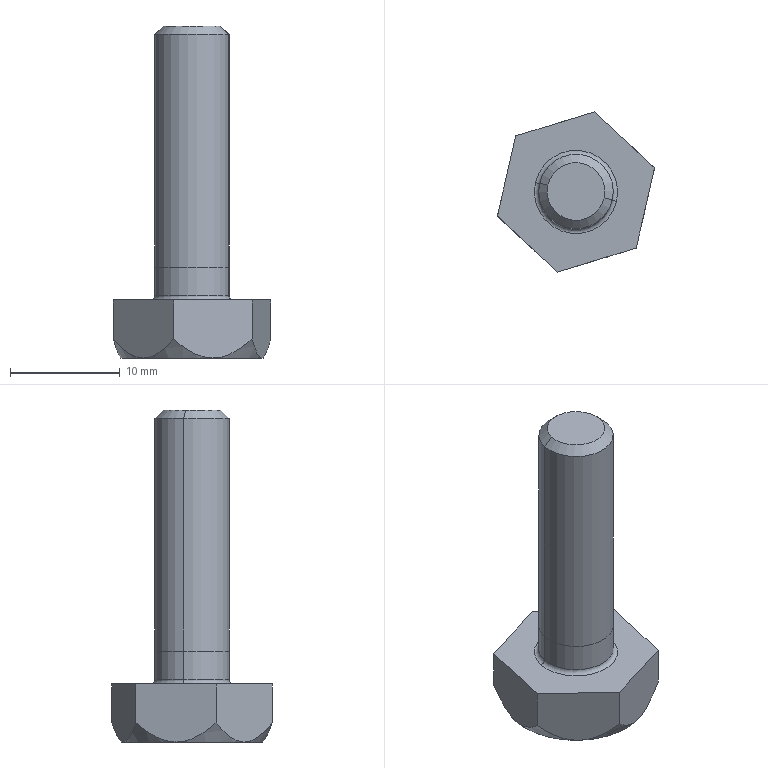Component | SolidWorks | Bolt-1 | 2 solids | 25 faces | box 14.35 x 14.63 x 30.3 mm | volume 1671 mm3 | plane 11 | cone 8 | cylinder 4 | torus 2 | commonest cylinder face diameters 6.8 x4
STEP:
#1=COLOUR_RGB('',0.7922,0.8196,0.9333);
#2=FILL_AREA_STYLE_COLOUR('',#1);
#3=FILL_AREA_STYLE('',(#2));
#4=SURFACE_STYLE_FILL_AREA(#3);
#5=SURFACE_SIDE_STYLE('',(#4));
#6=SURFACE_STYLE_USAGE(.BOTH.,#5);
#7=PRESENTATION_STYLE_ASSIGNMENT((#6));
#8=CARTESIAN_POINT('',(-1.433,1.919,3.87));
#9=VERTEX_POINT('',#8);
#10=CARTESIAN_POINT('',(-1.694,1.979,3.87));
#11=VERTEX_POINT('',#10);
#12=CARTESIAN_POINT('',(-1.564,1.949,3.87));
#13=DIRECTION('',(0.,0.,1.));
#14=DIRECTION('',(-0.9745,0.2245,0.));
#15=AXIS2_PLACEMENT_3D('',#12,#13,#14);
#16=CIRCLE('',#15,0.1339);
#17=EDGE_CURVE('',#9,#11,#16,.T.);
#18=ORIENTED_EDGE('',*,*,#17,.F.);
#19=CARTESIAN_POINT('',(-1.418,1.916,3.854));
#20=VERTEX_POINT('',#19);
#21=CARTESIAN_POINT('',(-1.418,1.916,3.87));
#22=DIRECTION('',(-0.2245,-0.9745,0.));
#23=DIRECTION('',(0.9745,-0.2245,0.));
#24=AXIS2_PLACEMENT_3D('',#21,#22,#23);
#25=CIRCLE('',#24,0.01575);
#26=EDGE_CURVE('',#9,#20,#25,.T.);
#27=ORIENTED_EDGE('',*,*,#26,.T.);
#28=CARTESIAN_POINT('',(-1.71,1.983,3.854));
#29=VERTEX_POINT('',#28);
#30=CARTESIAN_POINT('',(-1.564,1.949,3.854));
#31=DIRECTION('',(0.,0.,-1.));
#32=DIRECTION('',(-0.9745,0.2245,0.));
#33=AXIS2_PLACEMENT_3D('',#30,#31,#32);
#34=CIRCLE('',#33,0.1496);
#35=EDGE_CURVE('',#29,#20,#34,.T.);
#36=ORIENTED_EDGE('',*,*,#35,.F.);
#37=CARTESIAN_POINT('',(-1.71,1.983,3.87));
#38=DIRECTION('',(0.2245,0.9745,0.));
#39=DIRECTION('',(-0.9745,0.2245,0.));
#40=AXIS2_PLACEMENT_3D('',#37,#38,#39);
#41=CIRCLE('',#40,0.01575);
#42=EDGE_CURVE('',#11,#29,#41,.T.);
#43=ORIENTED_EDGE('',*,*,#42,.F.);
#44=EDGE_LOOP('',(#18,#27,#36,#43));
#45=FACE_OUTER_BOUND('',#44,.T.);
#46=CARTESIAN_POINT('',(-1.564,1.949,3.87));
#47=DIRECTION('',(0.,0.,1.));
#48=DIRECTION('',(-0.9745,0.2245,0.));
#49=AXIS2_PLACEMENT_3D('',#46,#47,#48);
#50=TOROIDAL_SURFACE('',#49,0.1496,0.01575);
#51=ADVANCED_FACE('',(#45),#50,.F.);
#52=CARTESIAN_POINT('',(-1.694,1.979,3.972));
#53=VERTEX_POINT('',#52);
#54=CARTESIAN_POINT('',(-1.433,1.919,3.972));
#55=VERTEX_POINT('',#54);
#56=CARTESIAN_POINT('',(-1.564,1.949,3.972));
#57=DIRECTION('',(0.,0.,1.));
#58=DIRECTION('',(-0.9745,0.2245,0.));
#59=AXIS2_PLACEMENT_3D('',#56,#57,#58);
#60=CIRCLE('',#59,0.1339);
#61=EDGE_CURVE('',#53,#55,#60,.T.);
#62=ORIENTED_EDGE('',*,*,#61,.F.);
#63=CARTESIAN_POINT('',(-1.694,1.979,3.972));
#64=DIRECTION('',(0.,0.,-1.));
#65=VECTOR('',#64,39.37);
#66=LINE('',#63,#65);
#67=EDGE_CURVE('',#53,#11,#66,.T.);
#68=ORIENTED_EDGE('',*,*,#67,.T.);
#69=CARTESIAN_POINT('',(-1.564,1.949,3.87));
#70=DIRECTION('',(0.,0.,1.));
#71=DIRECTION('',(-0.9745,0.2245,0.));
#72=AXIS2_PLACEMENT_3D('',#69,#70,#71);
#73=CIRCLE('',#72,0.1339);
#74=EDGE_CURVE('',#11,#9,#73,.T.);
#75=ORIENTED_EDGE('',*,*,#74,.T.);
#76=CARTESIAN_POINT('',(-1.433,1.919,3.972));
#77=DIRECTION('',(0.,0.,-1.));
#78=VECTOR('',#77,39.37);
#79=LINE('',#76,#78);
#80=EDGE_CURVE('',#55,#9,#79,.T.);
#81=ORIENTED_EDGE('',*,*,#80,.F.);
#82=EDGE_LOOP('',(#62,#68,#75,#81));
#83=FACE_OUTER_BOUND('',#82,.T.);
#84=CARTESIAN_POINT('',(-1.564,1.949,3.972));
#85=DIRECTION('',(0.,0.,-1.));
#86=DIRECTION('',(0.9745,-0.2245,0.));
#87=AXIS2_PLACEMENT_3D('',#84,#85,#86);
#88=CYLINDRICAL_SURFACE('',#87,0.1339);
#89=ADVANCED_FACE('',(#83),#88,.T.);
#90=CARTESIAN_POINT('',(-1.348,1.748,3.714));
#91=VERTEX_POINT('',#90);
#92=CARTESIAN_POINT('',(-1.489,1.705,3.646));
#93=VERTEX_POINT('',#92);
#94=CARTESIAN_POINT('',(-1.348,1.748,3.714));
#95=CARTESIAN_POINT('',(-1.358,1.745,3.705));
#96=CARTESIAN_POINT('',(-1.368,1.742,3.696));
#97=CARTESIAN_POINT('',(-1.389,1.735,3.681));
#98=CARTESIAN_POINT('',(-1.401,1.732,3.673));
#99=CARTESIAN_POINT('',(-1.424,1.725,3.66));
#100=CARTESIAN_POINT('',(-1.437,1.721,3.655));
#101=CARTESIAN_POINT('',(-1.456,1.715,3.65));
#102=CARTESIAN_POINT('',(-1.462,1.713,3.648));
#103=CARTESIAN_POINT('',(-1.475,1.709,3.646));
#104=CARTESIAN_POINT('',(-1.482,1.707,3.646));
#105=CARTESIAN_POINT('',(-1.489,1.705,3.646));
#106=B_SPLINE_CURVE_WITH_KNOTS('',3,(#94,#95,#96,#97,#98,#99,#100,#101,#102,#103,#104,#105),.UNSPECIFIED.,.F.,.F.,(4,2,2,2,2,4),(0.0000003,0.001051,0.002101,0.003151,0.003676,0.004201),.UNSPECIFIED.);
#107=EDGE_CURVE('',#91,#93,#106,.T.);
#108=ORIENTED_EDGE('',*,*,#107,.F.);
#109=CARTESIAN_POINT('',(-1.348,1.748,3.854));
#110=VERTEX_POINT('',#109);
#111=CARTESIAN_POINT('',(-1.348,1.748,3.854));
#112=DIRECTION('',(0.,0.,-1.));
#113=VECTOR('',#112,39.37);
#114=LINE('',#111,#113);
#115=EDGE_CURVE('',#110,#91,#114,.T.);
#116=ORIENTED_EDGE('',*,*,#115,.F.);
#117=CARTESIAN_POINT('',(-1.63,1.661,3.854));
#118=VERTEX_POINT('',#117);
#119=CARTESIAN_POINT('',(-1.63,1.661,3.854));
#120=DIRECTION('',(0.9562,0.2928,0.));
#121=VECTOR('',#120,39.37);
#122=LINE('',#119,#121);
#123=EDGE_CURVE('',#118,#110,#122,.T.);
#124=ORIENTED_EDGE('',*,*,#123,.F.);
#125=CARTESIAN_POINT('',(-1.63,1.661,3.714));
#126=VERTEX_POINT('',#125);
#127=CARTESIAN_POINT('',(-1.63,1.661,3.854));
#128=DIRECTION('',(0.,0.,-1.));
#129=VECTOR('',#128,39.37);
#130=LINE('',#127,#129);
#131=EDGE_CURVE('',#118,#126,#130,.T.);
#132=ORIENTED_EDGE('',*,*,#131,.T.);
#133=CARTESIAN_POINT('',(-1.489,1.705,3.646));
#134=CARTESIAN_POINT('',(-1.502,1.701,3.646));
#135=CARTESIAN_POINT('',(-1.515,1.697,3.648));
#136=CARTESIAN_POINT('',(-1.541,1.689,3.655));
#137=CARTESIAN_POINT('',(-1.553,1.685,3.66));
#138=CARTESIAN_POINT('',(-1.577,1.678,3.673));
#139=CARTESIAN_POINT('',(-1.588,1.674,3.68));
#140=CARTESIAN_POINT('',(-1.61,1.668,3.696));
#141=CARTESIAN_POINT('',(-1.62,1.665,3.705));
#142=CARTESIAN_POINT('',(-1.63,1.661,3.714));
#143=B_SPLINE_CURVE_WITH_KNOTS('',3,(#133,#134,#135,#136,#137,#138,#139,#140,#141,#142),.UNSPECIFIED.,.F.,.F.,(4,2,2,2,4),(0.004201,0.00525,0.006298,0.007347,0.008395),.UNSPECIFIED.);
#144=EDGE_CURVE('',#93,#126,#143,.T.);
#145=ORIENTED_EDGE('',*,*,#144,.F.);
#146=EDGE_LOOP('',(#108,#116,#124,#132,#145));
#147=FACE_OUTER_BOUND('',#146,.T.);
#148=CARTESIAN_POINT('',(-1.63,1.661,3.854));
#149=DIRECTION('',(-0.2928,0.9562,0.));
#150=DIRECTION('',(-0.9562,-0.2928,0.));
#151=AXIS2_PLACEMENT_3D('',#148,#149,#150);
#152=PLANE('',#151);
#153=ADVANCED_FACE('',(#147),#152,.F.);
#154=CARTESIAN_POINT('',(-1.281,2.036,3.714));
#155=VERTEX_POINT('',#154);
#156=CARTESIAN_POINT('',(-1.314,1.892,3.646));
#157=VERTEX_POINT('',#156);
#158=CARTESIAN_POINT('',(-1.281,2.036,3.714));
#159=CARTESIAN_POINT('',(-1.284,2.026,3.705));
#160=CARTESIAN_POINT('',(-1.286,2.015,3.697));
#161=CARTESIAN_POINT('',(-1.291,1.993,3.68));
#162=CARTESIAN_POINT('',(-1.294,1.982,3.673));
#163=CARTESIAN_POINT('',(-1.299,1.958,3.66));
#164=CARTESIAN_POINT('',(-1.302,1.945,3.655));
#165=CARTESIAN_POINT('',(-1.307,1.925,3.65));
#166=CARTESIAN_POINT('',(-1.308,1.919,3.648));
#167=CARTESIAN_POINT('',(-1.311,1.905,3.646));
#168=CARTESIAN_POINT('',(-1.313,1.899,3.646));
#169=CARTESIAN_POINT('',(-1.314,1.892,3.646));
#170=B_SPLINE_CURVE_WITH_KNOTS('',3,(#158,#159,#160,#161,#162,#163,#164,#165,#166,#167,#168,#169),.UNSPECIFIED.,.F.,.F.,(4,2,2,2,2,4),(0.01522,0.01628,0.01734,0.01839,0.01892,0.01945),.UNSPECIFIED.);
#171=EDGE_CURVE('',#155,#157,#170,.T.);
#172=ORIENTED_EDGE('',*,*,#171,.F.);
#173=CARTESIAN_POINT('',(-1.281,2.036,3.854));
#174=VERTEX_POINT('',#173);
#175=CARTESIAN_POINT('',(-1.281,2.036,3.854));
#176=DIRECTION('',(0.,0.,-1.));
#177=VECTOR('',#176,39.37);
#178=LINE('',#175,#177);
#179=EDGE_CURVE('',#174,#155,#178,.T.);
#180=ORIENTED_EDGE('',*,*,#179,.F.);
#181=CARTESIAN_POINT('',(-1.348,1.748,3.854));
#182=DIRECTION('',(0.2245,0.9745,0.));
#183=VECTOR('',#182,39.37);
#184=LINE('',#181,#183);
#185=EDGE_CURVE('',#110,#174,#184,.T.);
#186=ORIENTED_EDGE('',*,*,#185,.F.);
#187=ORIENTED_EDGE('',*,*,#115,.T.);
#188=CARTESIAN_POINT('',(-1.314,1.892,3.646));
#189=CARTESIAN_POINT('',(-1.316,1.885,3.646));
#190=CARTESIAN_POINT('',(-1.317,1.879,3.646));
#191=CARTESIAN_POINT('',(-1.321,1.865,3.648));
#192=CARTESIAN_POINT('',(-1.322,1.858,3.65));
#193=CARTESIAN_POINT('',(-1.327,1.839,3.655));
#194=CARTESIAN_POINT('',(-1.33,1.826,3.66));
#195=CARTESIAN_POINT('',(-1.335,1.802,3.673));
#196=CARTESIAN_POINT('',(-1.338,1.791,3.681));
#197=CARTESIAN_POINT('',(-1.343,1.769,3.697));
#198=CARTESIAN_POINT('',(-1.345,1.758,3.705));
#199=CARTESIAN_POINT('',(-1.348,1.748,3.714));
#200=B_SPLINE_CURVE_WITH_KNOTS('',3,(#188,#189,#190,#191,#192,#193,#194,#195,#196,#197,#198,#199),.UNSPECIFIED.,.F.,.F.,(4,2,2,2,2,4),(0.01945,0.01998,0.02051,0.02157,0.02263,0.02369),.UNSPECIFIED.);
#201=EDGE_CURVE('',#157,#91,#200,.T.);
#202=ORIENTED_EDGE('',*,*,#201,.F.);
#203=EDGE_LOOP('',(#172,#180,#186,#187,#202));
#204=FACE_OUTER_BOUND('',#203,.T.);
#205=CARTESIAN_POINT('',(-1.348,1.748,3.854));
#206=DIRECTION('',(-0.9745,0.2245,0.));
#207=DIRECTION('',(0.,0.,-1.));
#208=AXIS2_PLACEMENT_3D('',#205,#206,#207);
#209=PLANE('',#208);
#210=ADVANCED_FACE('',(#204),#209,.F.);
#211=CARTESIAN_POINT('',(-1.497,2.237,3.714));
#212=VERTEX_POINT('',#211);
#213=CARTESIAN_POINT('',(-1.389,2.137,3.646));
#214=VERTEX_POINT('',#213);
#215=CARTESIAN_POINT('',(-1.497,2.237,3.714));
#216=CARTESIAN_POINT('',(-1.49,2.23,3.705));
#217=CARTESIAN_POINT('',(-1.482,2.223,3.696));
#218=CARTESIAN_POINT('',(-1.465,2.207,3.681));
#219=CARTESIAN_POINT('',(-1.457,2.2,3.673));
#220=CARTESIAN_POINT('',(-1.439,2.183,3.66));
#221=CARTESIAN_POINT('',(-1.429,2.174,3.655));
#222=CARTESIAN_POINT('',(-1.415,2.16,3.65));
#223=CARTESIAN_POINT('',(-1.41,2.156,3.648));
#224=CARTESIAN_POINT('',(-1.4,2.146,3.646));
#225=CARTESIAN_POINT('',(-1.394,2.141,3.646));
#226=CARTESIAN_POINT('',(-1.389,2.137,3.646));
#227=B_SPLINE_CURVE_WITH_KNOTS('',3,(#215,#216,#217,#218,#219,#220,#221,#222,#223,#224,#225,#226),.UNSPECIFIED.,.F.,.F.,(4,2,2,2,2,4),(0.0000003,0.001051,0.002101,0.003151,0.003676,0.004201),.UNSPECIFIED.);
#228=EDGE_CURVE('',#212,#214,#227,.T.);
#229=ORIENTED_EDGE('',*,*,#228,.F.);
#230=CARTESIAN_POINT('',(-1.497,2.237,3.854));
#231=VERTEX_POINT('',#230);
#232=CARTESIAN_POINT('',(-1.497,2.237,3.854));
#233=DIRECTION('',(0.,0.,-1.));
#234=VECTOR('',#233,39.37);
#235=LINE('',#232,#234);
#236=EDGE_CURVE('',#231,#212,#235,.T.);
#237=ORIENTED_EDGE('',*,*,#236,.F.);
#238=CARTESIAN_POINT('',(-1.281,2.036,3.854));
#239=DIRECTION('',(-0.7317,0.6817,0.));
#240=VECTOR('',#239,39.37);
#241=LINE('',#238,#240);
#242=EDGE_CURVE('',#174,#231,#241,.T.);
#243=ORIENTED_EDGE('',*,*,#242,.F.);
#244=ORIENTED_EDGE('',*,*,#179,.T.);
#245=CARTESIAN_POINT('',(-1.389,2.137,3.646));
#246=CARTESIAN_POINT('',(-1.379,2.127,3.646));
#247=CARTESIAN_POINT('',(-1.369,2.118,3.648));
#248=CARTESIAN_POINT('',(-1.349,2.099,3.655));
#249=CARTESIAN_POINT('',(-1.34,2.091,3.66));
#250=CARTESIAN_POINT('',(-1.322,2.074,3.673));
#251=CARTESIAN_POINT('',(-1.313,2.066,3.68));
#252=CARTESIAN_POINT('',(-1.297,2.05,3.696));
#253=CARTESIAN_POINT('',(-1.289,2.043,3.705));
#254=CARTESIAN_POINT('',(-1.281,2.036,3.714));
#255=B_SPLINE_CURVE_WITH_KNOTS('',3,(#245,#246,#247,#248,#249,#250,#251,#252,#253,#254),.UNSPECIFIED.,.F.,.F.,(4,2,2,2,4),(0.004201,0.00525,0.006298,0.007347,0.008395),.UNSPECIFIED.);
#256=EDGE_CURVE('',#214,#155,#255,.T.);
#257=ORIENTED_EDGE('',*,*,#256,.F.);
#258=EDGE_LOOP('',(#229,#237,#243,#244,#257));
#259=FACE_OUTER_BOUND('',#258,.T.);
#260=CARTESIAN_POINT('',(-1.281,2.036,3.854));
#261=DIRECTION('',(-0.6817,-0.7317,0.));
#262=DIRECTION('',(0.7317,-0.6817,0.));
#263=AXIS2_PLACEMENT_3D('',#260,#261,#262);
#264=PLANE('',#263);
#265=ADVANCED_FACE('',(#259),#264,.F.);
#266=CARTESIAN_POINT('',(-1.78,2.151,3.714));
#267=VERTEX_POINT('',#266);
#268=CARTESIAN_POINT('',(-1.639,2.194,3.646));
#269=VERTEX_POINT('',#268);
#270=CARTESIAN_POINT('',(-1.78,2.151,3.714));
#271=CARTESIAN_POINT('',(-1.77,2.154,3.705));
#272=CARTESIAN_POINT('',(-1.76,2.157,3.696));
#273=CARTESIAN_POINT('',(-1.738,2.164,3.681));
#274=CARTESIAN_POINT('',(-1.727,2.167,3.673));
#275=CARTESIAN_POINT('',(-1.703,2.174,3.66));
#276=CARTESIAN_POINT('',(-1.691,2.178,3.655));
#277=CARTESIAN_POINT('',(-1.672,2.184,3.65));
#278=CARTESIAN_POINT('',(-1.665,2.186,3.648));
#279=CARTESIAN_POINT('',(-1.652,2.19,3.646));
#280=CARTESIAN_POINT('',(-1.645,2.192,3.646));
#281=CARTESIAN_POINT('',(-1.639,2.194,3.646));
#282=B_SPLINE_CURVE_WITH_KNOTS('',3,(#270,#271,#272,#273,#274,#275,#276,#277,#278,#279,#280,#281),.UNSPECIFIED.,.F.,.F.,(4,2,2,2,2,4),(0.0000003,0.001051,0.002101,0.003151,0.003676,0.004201),.UNSPECIFIED.);
#283=EDGE_CURVE('',#267,#269,#282,.T.);
#284=ORIENTED_EDGE('',*,*,#283,.F.);
#285=CARTESIAN_POINT('',(-1.78,2.151,3.854));
#286=VERTEX_POINT('',#285);
#287=CARTESIAN_POINT('',(-1.78,2.151,3.854));
#288=DIRECTION('',(0.,0.,-1.));
#289=VECTOR('',#288,39.37);
#290=LINE('',#287,#289);
#291=EDGE_CURVE('',#286,#267,#290,.T.);
#292=ORIENTED_EDGE('',*,*,#291,.F.);
#293=CARTESIAN_POINT('',(-1.497,2.237,3.854));
#294=DIRECTION('',(-0.9562,-0.2928,0.));
#295=VECTOR('',#294,39.37);
#296=LINE('',#293,#295);
#297=EDGE_CURVE('',#231,#286,#296,.T.);
#298=ORIENTED_EDGE('',*,*,#297,.F.);
#299=ORIENTED_EDGE('',*,*,#236,.T.);
#300=CARTESIAN_POINT('',(-1.639,2.194,3.646));
#301=CARTESIAN_POINT('',(-1.625,2.198,3.646));
#302=CARTESIAN_POINT('',(-1.612,2.202,3.648));
#303=CARTESIAN_POINT('',(-1.587,2.21,3.655));
#304=CARTESIAN_POINT('',(-1.574,2.214,3.66));
#305=CARTESIAN_POINT('',(-1.551,2.221,3.673));
#306=CARTESIAN_POINT('',(-1.54,2.224,3.68));
#307=CARTESIAN_POINT('',(-1.518,2.231,3.696));
#308=CARTESIAN_POINT('',(-1.507,2.234,3.705));
#309=CARTESIAN_POINT('',(-1.497,2.237,3.714));
#310=B_SPLINE_CURVE_WITH_KNOTS('',3,(#300,#301,#302,#303,#304,#305,#306,#307,#308,#309),.UNSPECIFIED.,.F.,.F.,(4,2,2,2,4),(0.004201,0.00525,0.006298,0.007347,0.008395),.UNSPECIFIED.);
#311=EDGE_CURVE('',#269,#212,#310,.T.);
#312=ORIENTED_EDGE('',*,*,#311,.F.);
#313=EDGE_LOOP('',(#284,#292,#298,#299,#312));
#314=FACE_OUTER_BOUND('',#313,.T.);
#315=CARTESIAN_POINT('',(-1.497,2.237,3.854));
#316=DIRECTION('',(0.2928,-0.9562,0.));
#317=DIRECTION('',(0.9562,0.2928,0.));
#318=AXIS2_PLACEMENT_3D('',#315,#316,#317);
#319=PLANE('',#318);
#320=ADVANCED_FACE('',(#314),#319,.F.);
#321=CARTESIAN_POINT('',(-1.846,1.863,3.714));
#322=VERTEX_POINT('',#321);
#323=CARTESIAN_POINT('',(-1.813,2.007,3.646));
#324=VERTEX_POINT('',#323);
#325=CARTESIAN_POINT('',(-1.846,1.863,3.714));
#326=CARTESIAN_POINT('',(-1.844,1.873,3.705));
#327=CARTESIAN_POINT('',(-1.842,1.884,3.697));
#328=CARTESIAN_POINT('',(-1.836,1.906,3.68));
#329=CARTESIAN_POINT('',(-1.834,1.917,3.673));
#330=CARTESIAN_POINT('',(-1.828,1.941,3.66));
#331=CARTESIAN_POINT('',(-1.825,1.954,3.655));
#332=CARTESIAN_POINT('',(-1.821,1.973,3.65));
#333=CARTESIAN_POINT('',(-1.819,1.98,3.648));
#334=CARTESIAN_POINT('',(-1.816,1.993,3.646));
#335=CARTESIAN_POINT('',(-1.815,2.,3.646));
#336=CARTESIAN_POINT('',(-1.813,2.007,3.646));
#337=B_SPLINE_CURVE_WITH_KNOTS('',3,(#325,#326,#327,#328,#329,#330,#331,#332,#333,#334,#335,#336),.UNSPECIFIED.,.F.,.F.,(4,2,2,2,2,4),(0.01522,0.01628,0.01734,0.01839,0.01892,0.01945),.UNSPECIFIED.);
#338=EDGE_CURVE('',#322,#324,#337,.T.);
#339=ORIENTED_EDGE('',*,*,#338,.F.);
#340=CARTESIAN_POINT('',(-1.846,1.863,3.854));
#341=VERTEX_POINT('',#340);
#342=CARTESIAN_POINT('',(-1.846,1.863,3.854));
#343=DIRECTION('',(0.,0.,-1.));
#344=VECTOR('',#343,39.37);
#345=LINE('',#342,#344);
#346=EDGE_CURVE('',#341,#322,#345,.T.);
#347=ORIENTED_EDGE('',*,*,#346,.F.);
#348=CARTESIAN_POINT('',(-1.78,2.151,3.854));
#349=DIRECTION('',(-0.2245,-0.9745,0.));
#350=VECTOR('',#349,39.37);
#351=LINE('',#348,#350);
#352=EDGE_CURVE('',#286,#341,#351,.T.);
#353=ORIENTED_EDGE('',*,*,#352,.F.);
#354=ORIENTED_EDGE('',*,*,#291,.T.);
#355=CARTESIAN_POINT('',(-1.813,2.007,3.646));
#356=CARTESIAN_POINT('',(-1.812,2.014,3.646));
#357=CARTESIAN_POINT('',(-1.81,2.02,3.646));
#358=CARTESIAN_POINT('',(-1.807,2.034,3.648));
#359=CARTESIAN_POINT('',(-1.805,2.04,3.65));
#360=CARTESIAN_POINT('',(-1.801,2.06,3.655));
#361=CARTESIAN_POINT('',(-1.798,2.073,3.66));
#362=CARTESIAN_POINT('',(-1.792,2.097,3.673));
#363=CARTESIAN_POINT('',(-1.79,2.108,3.681));
#364=CARTESIAN_POINT('',(-1.785,2.13,3.697));
#365=CARTESIAN_POINT('',(-1.782,2.141,3.705));
#366=CARTESIAN_POINT('',(-1.78,2.151,3.714));
#367=B_SPLINE_CURVE_WITH_KNOTS('',3,(#355,#356,#357,#358,#359,#360,#361,#362,#363,#364,#365,#366),.UNSPECIFIED.,.F.,.F.,(4,2,2,2,2,4),(0.01945,0.01998,0.02051,0.02157,0.02263,0.02369),.UNSPECIFIED.);
#368=EDGE_CURVE('',#324,#267,#367,.T.);
#369=ORIENTED_EDGE('',*,*,#368,.F.);
#370=EDGE_LOOP('',(#339,#347,#353,#354,#369));
#371=FACE_OUTER_BOUND('',#370,.T.);
#372=CARTESIAN_POINT('',(-1.78,2.151,3.854));
#373=DIRECTION('',(0.9745,-0.2245,0.));
#374=DIRECTION('',(0.2245,0.9745,0.));
#375=AXIS2_PLACEMENT_3D('',#372,#373,#374);
#376=PLANE('',#375);
#377=ADVANCED_FACE('',(#371),#376,.F.);
#378=CARTESIAN_POINT('',(-1.738,1.762,3.646));
#379=VERTEX_POINT('',#378);
#380=CARTESIAN_POINT('',(-1.63,1.661,3.714));
#381=CARTESIAN_POINT('',(-1.638,1.669,3.705));
#382=CARTESIAN_POINT('',(-1.646,1.676,3.696));
#383=CARTESIAN_POINT('',(-1.662,1.691,3.681));
#384=CARTESIAN_POINT('',(-1.671,1.699,3.673));
#385=CARTESIAN_POINT('',(-1.689,1.716,3.66));
#386=CARTESIAN_POINT('',(-1.698,1.725,3.655));
#387=CARTESIAN_POINT('',(-1.713,1.739,3.65));
#388=CARTESIAN_POINT('',(-1.718,1.743,3.648));
#389=CARTESIAN_POINT('',(-1.728,1.753,3.646));
#390=CARTESIAN_POINT('',(-1.733,1.757,3.646));
#391=CARTESIAN_POINT('',(-1.738,1.762,3.646));
#392=B_SPLINE_CURVE_WITH_KNOTS('',3,(#380,#381,#382,#383,#384,#385,#386,#387,#388,#389,#390,#391),.UNSPECIFIED.,.F.,.F.,(4,2,2,2,2,4),(0.0000003,0.001051,0.002101,0.003151,0.003676,0.004201),.UNSPECIFIED.);
#393=EDGE_CURVE('',#126,#379,#392,.T.);
#394=ORIENTED_EDGE('',*,*,#393,.F.);
#395=ORIENTED_EDGE('',*,*,#131,.F.);
#396=CARTESIAN_POINT('',(-1.846,1.863,3.854));
#397=DIRECTION('',(0.7317,-0.6817,0.));
#398=VECTOR('',#397,39.37);
#399=LINE('',#396,#398);
#400=EDGE_CURVE('',#341,#118,#399,.T.);
#401=ORIENTED_EDGE('',*,*,#400,.F.);
#402=ORIENTED_EDGE('',*,*,#346,.T.);
#403=CARTESIAN_POINT('',(-1.738,1.762,3.646));
#404=CARTESIAN_POINT('',(-1.748,1.772,3.646));
#405=CARTESIAN_POINT('',(-1.758,1.781,3.648));
#406=CARTESIAN_POINT('',(-1.778,1.799,3.655));
#407=CARTESIAN_POINT('',(-1.787,1.808,3.66));
#408=CARTESIAN_POINT('',(-1.805,1.825,3.673));
#409=CARTESIAN_POINT('',(-1.814,1.833,3.68));
#410=CARTESIAN_POINT('',(-1.831,1.848,3.696));
#411=CARTESIAN_POINT('',(-1.839,1.856,3.705));
#412=CARTESIAN_POINT('',(-1.846,1.863,3.714));
#413=B_SPLINE_CURVE_WITH_KNOTS('',3,(#403,#404,#405,#406,#407,#408,#409,#410,#411,#412),.UNSPECIFIED.,.F.,.F.,(4,2,2,2,4),(0.004201,0.00525,0.006298,0.007347,0.008395),.UNSPECIFIED.);
#414=EDGE_CURVE('',#379,#322,#413,.T.);
#415=ORIENTED_EDGE('',*,*,#414,.F.);
#416=EDGE_LOOP('',(#394,#395,#401,#402,#415));
#417=FACE_OUTER_BOUND('',#416,.T.);
#418=CARTESIAN_POINT('',(-1.846,1.863,3.854));
#419=DIRECTION('',(0.6817,0.7317,0.));
#420=DIRECTION('',(-0.7317,0.6817,0.));
#421=AXIS2_PLACEMENT_3D('',#418,#419,#420);
#422=PLANE('',#421);
#423=ADVANCED_FACE('',(#417),#422,.F.);
#424=ORIENTED_EDGE('',*,*,#35,.T.);
#425=CARTESIAN_POINT('',(-1.564,1.949,3.854));
#426=DIRECTION('',(0.,0.,-1.));
#427=DIRECTION('',(-0.9745,0.2245,0.));
#428=AXIS2_PLACEMENT_3D('',#425,#426,#427);
#429=CIRCLE('',#428,0.1496);
#430=EDGE_CURVE('',#20,#29,#429,.T.);
#431=ORIENTED_EDGE('',*,*,#430,.T.);
#432=EDGE_LOOP('',(#424,#431));
#433=FACE_BOUND('',#432,.T.);
#434=ORIENTED_EDGE('',*,*,#123,.T.);
#435=ORIENTED_EDGE('',*,*,#185,.T.);
#436=ORIENTED_EDGE('',*,*,#242,.T.);
#437=ORIENTED_EDGE('',*,*,#297,.T.);
#438=ORIENTED_EDGE('',*,*,#352,.T.);
#439=ORIENTED_EDGE('',*,*,#400,.T.);
#440=EDGE_LOOP('',(#434,#435,#436,#437,#438,#439));
#441=FACE_OUTER_BOUND('',#440,.T.);
#442=CARTESIAN_POINT('',(-1.564,1.949,3.854));
#443=DIRECTION('',(0.,0.,1.));
#444=DIRECTION('',(-0.9745,0.2245,0.));
#445=AXIS2_PLACEMENT_3D('',#442,#443,#444);
#446=PLANE('',#445);
#447=ADVANCED_FACE('',(#433,#441),#446,.T.);
#448=ORIENTED_EDGE('',*,*,#67,.F.);
#449=CARTESIAN_POINT('',(-1.564,1.949,3.972));
#450=DIRECTION('',(0.,0.,1.));
#451=DIRECTION('',(-0.9745,0.2245,0.));
#452=AXIS2_PLACEMENT_3D('',#449,#450,#451);
#453=CIRCLE('',#452,0.1339);
#454=EDGE_CURVE('',#55,#53,#453,.T.);
#455=ORIENTED_EDGE('',*,*,#454,.F.);
#456=ORIENTED_EDGE('',*,*,#80,.T.);
#457=ORIENTED_EDGE('',*,*,#17,.T.);
#458=EDGE_LOOP('',(#448,#455,#456,#457));
#459=FACE_OUTER_BOUND('',#458,.T.);
#460=CARTESIAN_POINT('',(-1.564,1.949,3.972));
#461=DIRECTION('',(0.,0.,-1.));
#462=DIRECTION('',(0.9745,-0.2245,0.));
#463=AXIS2_PLACEMENT_3D('',#460,#461,#462);
#464=CYLINDRICAL_SURFACE('',#463,0.1339);
#465=ADVANCED_FACE('',(#459),#464,.T.);
#466=ORIENTED_EDGE('',*,*,#454,.T.);
#467=ORIENTED_EDGE('',*,*,#61,.T.);
#468=EDGE_LOOP('',(#466,#467));
#469=FACE_OUTER_BOUND('',#468,.T.);
#470=CARTESIAN_POINT('',(-1.564,1.949,3.972));
#471=DIRECTION('',(0.,0.,1.));
#472=DIRECTION('',(-0.9745,0.2245,0.));
#473=AXIS2_PLACEMENT_3D('',#470,#471,#472);
#474=PLANE('',#473);
#475=ADVANCED_FACE('',(#469),#474,.T.);
#476=ORIENTED_EDGE('',*,*,#26,.F.);
#477=ORIENTED_EDGE('',*,*,#74,.F.);
#478=ORIENTED_EDGE('',*,*,#42,.T.);
#479=ORIENTED_EDGE('',*,*,#430,.F.);
#480=EDGE_LOOP('',(#476,#477,#478,#479));
#481=FACE_OUTER_BOUND('',#480,.T.);
#482=CARTESIAN_POINT('',(-1.564,1.949,3.87));
#483=DIRECTION('',(0.,0.,1.));
#484=DIRECTION('',(-0.9745,0.2245,0.));
#485=AXIS2_PLACEMENT_3D('',#482,#483,#484);
#486=TOROIDAL_SURFACE('',#485,0.1496,0.01575);
#487=ADVANCED_FACE('',(#481),#486,.F.);
#488=ORIENTED_EDGE('',*,*,#283,.T.);
#489=CARTESIAN_POINT('',(-1.564,1.949,3.646));
#490=DIRECTION('',(0.,0.,1.));
#491=DIRECTION('',(-0.9745,0.2245,0.));
#492=AXIS2_PLACEMENT_3D('',#489,#490,#491);
#493=CIRCLE('',#492,0.2559);
#494=EDGE_CURVE('',#269,#324,#493,.T.);
#495=ORIENTED_EDGE('',*,*,#494,.T.);
#496=ORIENTED_EDGE('',*,*,#368,.T.);
#497=EDGE_LOOP('',(#488,#495,#496));
#498=FACE_OUTER_BOUND('',#497,.T.);
#499=CARTESIAN_POINT('',(-1.564,1.949,3.646));
#500=DIRECTION('',(0.,0.,1.));
#501=DIRECTION('',(0.9745,-0.2245,0.));
#502=AXIS2_PLACEMENT_3D('',#499,#500,#501);
#503=CONICAL_SURFACE('',#502,0.2559,0.5236);
#504=ADVANCED_FACE('',(#498),#503,.T.);
#505=ORIENTED_EDGE('',*,*,#228,.T.);
#506=CARTESIAN_POINT('',(-1.564,1.949,3.646));
#507=DIRECTION('',(0.,0.,1.));
#508=DIRECTION('',(-0.9745,0.2245,0.));
#509=AXIS2_PLACEMENT_3D('',#506,#507,#508);
#510=CIRCLE('',#509,0.2559);
#511=EDGE_CURVE('',#214,#269,#510,.T.);
#512=ORIENTED_EDGE('',*,*,#511,.T.);
#513=ORIENTED_EDGE('',*,*,#311,.T.);
#514=EDGE_LOOP('',(#505,#512,#513));
#515=FACE_OUTER_BOUND('',#514,.T.);
#516=CARTESIAN_POINT('',(-1.564,1.949,3.646));
#517=DIRECTION('',(0.,0.,1.));
#518=DIRECTION('',(0.9745,-0.2245,0.));
#519=AXIS2_PLACEMENT_3D('',#516,#517,#518);
#520=CONICAL_SURFACE('',#519,0.2559,0.5236);
#521=ADVANCED_FACE('',(#515),#520,.T.);
#522=ORIENTED_EDGE('',*,*,#256,.T.);
#523=ORIENTED_EDGE('',*,*,#171,.T.);
#524=CARTESIAN_POINT('',(-1.564,1.949,3.646));
#525=DIRECTION('',(0.,0.,1.));
#526=DIRECTION('',(-0.9745,0.2245,0.));
#527=AXIS2_PLACEMENT_3D('',#524,#525,#526);
#528=CIRCLE('',#527,0.2559);
#529=EDGE_CURVE('',#157,#214,#528,.T.);
#530=ORIENTED_EDGE('',*,*,#529,.T.);
#531=EDGE_LOOP('',(#522,#523,#530));
#532=FACE_OUTER_BOUND('',#531,.T.);
#533=CARTESIAN_POINT('',(-1.564,1.949,3.646));
#534=DIRECTION('',(0.,0.,1.));
#535=DIRECTION('',(0.9745,-0.2245,0.));
#536=AXIS2_PLACEMENT_3D('',#533,#534,#535);
#537=CONICAL_SURFACE('',#536,0.2559,0.5236);
#538=ADVANCED_FACE('',(#532),#537,.T.);
#539=ORIENTED_EDGE('',*,*,#201,.T.);
#540=ORIENTED_EDGE('',*,*,#107,.T.);
#541=CARTESIAN_POINT('',(-1.564,1.949,3.646));
#542=DIRECTION('',(0.,0.,-1.));
#543=DIRECTION('',(0.9745,-0.2245,0.));
#544=AXIS2_PLACEMENT_3D('',#541,#542,#543);
#545=CIRCLE('',#544,0.2559);
#546=EDGE_CURVE('',#157,#93,#545,.T.);
#547=ORIENTED_EDGE('',*,*,#546,.F.);
#548=EDGE_LOOP('',(#539,#540,#547));
#549=FACE_OUTER_BOUND('',#548,.T.);
#550=CARTESIAN_POINT('',(-1.564,1.949,3.646));
#551=DIRECTION('',(0.,0.,1.));
#552=DIRECTION('',(0.9745,-0.2245,0.));
#553=AXIS2_PLACEMENT_3D('',#550,#551,#552);
#554=CONICAL_SURFACE('',#553,0.2559,0.5236);
#555=ADVANCED_FACE('',(#549),#554,.T.);
#556=ORIENTED_EDGE('',*,*,#144,.T.);
#557=ORIENTED_EDGE('',*,*,#393,.T.);
#558=CARTESIAN_POINT('',(-1.564,1.949,3.646));
#559=DIRECTION('',(0.,0.,1.));
#560=DIRECTION('',(-0.9745,0.2245,0.));
#561=AXIS2_PLACEMENT_3D('',#558,#559,#560);
#562=CIRCLE('',#561,0.2559);
#563=EDGE_CURVE('',#379,#93,#562,.T.);
#564=ORIENTED_EDGE('',*,*,#563,.T.);
#565=EDGE_LOOP('',(#556,#557,#564));
#566=FACE_OUTER_BOUND('',#565,.T.);
#567=CARTESIAN_POINT('',(-1.564,1.949,3.646));
#568=DIRECTION('',(0.,0.,1.));
#569=DIRECTION('',(0.9745,-0.2245,0.));
#570=AXIS2_PLACEMENT_3D('',#567,#568,#569);
#571=CONICAL_SURFACE('',#570,0.2559,0.5236);
#572=ADVANCED_FACE('',(#566),#571,.T.);
#573=ORIENTED_EDGE('',*,*,#338,.T.);
#574=CARTESIAN_POINT('',(-1.564,1.949,3.646));
#575=DIRECTION('',(0.,0.,1.));
#576=DIRECTION('',(-0.9745,0.2245,0.));
#577=AXIS2_PLACEMENT_3D('',#574,#575,#576);
#578=CIRCLE('',#577,0.2559);
#579=EDGE_CURVE('',#324,#379,#578,.T.);
#580=ORIENTED_EDGE('',*,*,#579,.T.);
#581=ORIENTED_EDGE('',*,*,#414,.T.);
#582=EDGE_LOOP('',(#573,#580,#581));
#583=FACE_OUTER_BOUND('',#582,.T.);
#584=CARTESIAN_POINT('',(-1.564,1.949,3.646));
#585=DIRECTION('',(0.,0.,1.));
#586=DIRECTION('',(0.9745,-0.2245,0.));
#587=AXIS2_PLACEMENT_3D('',#584,#585,#586);
#588=CONICAL_SURFACE('',#587,0.2559,0.5236);
#589=ADVANCED_FACE('',(#583),#588,.T.);
#590=ORIENTED_EDGE('',*,*,#579,.F.);
#591=ORIENTED_EDGE('',*,*,#494,.F.);
#592=ORIENTED_EDGE('',*,*,#511,.F.);
#593=ORIENTED_EDGE('',*,*,#529,.F.);
#594=ORIENTED_EDGE('',*,*,#546,.T.);
#595=ORIENTED_EDGE('',*,*,#563,.F.);
#596=EDGE_LOOP('',(#590,#591,#592,#593,#594,#595));
#597=FACE_OUTER_BOUND('',#596,.T.);
#598=CARTESIAN_POINT('',(-1.564,1.949,3.646));
#599=DIRECTION('',(0.,0.,1.));
#600=DIRECTION('',(-0.9745,0.2245,0.));
#601=AXIS2_PLACEMENT_3D('',#598,#599,#600);
#602=PLANE('',#601);
#603=ADVANCED_FACE('',(#597),#602,.F.);
#604=CLOSED_SHELL('',(#51,#89,#153,#210,#265,#320,#377,#423,#447,#465,#475,#487,#504,#521,#538,#555,#572,#589,#603));
#605=MANIFOLD_SOLID_BREP('',#604);
#606=STYLED_ITEM('',(#7),#605);
#607=PRESENTATION_LAYER_ASSIGNMENT('','',(#606));
#608=COLOUR_RGB('',0.7922,0.8196,0.9333);
#609=FILL_AREA_STYLE_COLOUR('',#608);
#610=FILL_AREA_STYLE('',(#609));
#611=SURFACE_STYLE_FILL_AREA(#610);
#612=SURFACE_SIDE_STYLE('',(#611));
#613=SURFACE_STYLE_USAGE(.BOTH.,#612);
#614=PRESENTATION_STYLE_ASSIGNMENT((#613));
#615=CARTESIAN_POINT('',(-1.665,1.973,4.839));
#616=VERTEX_POINT('',#615);
#617=CARTESIAN_POINT('',(-1.463,1.926,4.839));
#618=VERTEX_POINT('',#617);
#619=CARTESIAN_POINT('',(-1.564,1.949,4.839));
#620=DIRECTION('',(0.,0.,1.));
#621=DIRECTION('',(-0.9745,0.2245,0.));
#622=AXIS2_PLACEMENT_3D('',#619,#620,#621);
#623=CIRCLE('',#622,0.1035);
#624=EDGE_CURVE('',#616,#618,#623,.T.);
#625=ORIENTED_EDGE('',*,*,#624,.F.);
#626=CARTESIAN_POINT('',(-1.694,1.979,4.808));
#627=VERTEX_POINT('',#626);
#628=CARTESIAN_POINT('',(-1.665,1.973,4.839));
#629=DIRECTION('',(-0.6891,0.1587,-0.7071));
#630=VECTOR('',#629,39.37);
#631=LINE('',#628,#630);
#632=EDGE_CURVE('',#616,#627,#631,.T.);
#633=ORIENTED_EDGE('',*,*,#632,.T.);
#634=CARTESIAN_POINT('',(-1.433,1.919,4.808));
#635=VERTEX_POINT('',#634);
#636=CARTESIAN_POINT('',(-1.564,1.949,4.808));
#637=DIRECTION('',(0.,0.,-1.));
#638=DIRECTION('',(-0.9745,0.2245,0.));
#639=AXIS2_PLACEMENT_3D('',#636,#637,#638);
#640=CIRCLE('',#639,0.1339);
#641=EDGE_CURVE('',#635,#627,#640,.T.);
#642=ORIENTED_EDGE('',*,*,#641,.F.);
#643=CARTESIAN_POINT('',(-1.463,1.926,4.839));
#644=DIRECTION('',(0.6891,-0.1587,-0.7071));
#645=VECTOR('',#644,39.37);
#646=LINE('',#643,#645);
#647=EDGE_CURVE('',#618,#635,#646,.T.);
#648=ORIENTED_EDGE('',*,*,#647,.F.);
#649=EDGE_LOOP('',(#625,#633,#642,#648));
#650=FACE_OUTER_BOUND('',#649,.T.);
#651=CARTESIAN_POINT('',(-1.564,1.949,4.839));
#652=DIRECTION('',(0.,0.,-1.));
#653=DIRECTION('',(0.9745,-0.2245,0.));
#654=AXIS2_PLACEMENT_3D('',#651,#652,#653);
#655=CONICAL_SURFACE('',#654,0.1035,0.7854);
#656=ADVANCED_FACE('',(#650),#655,.T.);
#657=ORIENTED_EDGE('',*,*,#641,.T.);
#658=CARTESIAN_POINT('',(-1.694,1.979,3.972));
#659=VERTEX_POINT('',#658);
#660=CARTESIAN_POINT('',(-1.694,1.979,4.839));
#661=DIRECTION('',(0.,0.,-1.));
#662=VECTOR('',#661,39.37);
#663=LINE('',#660,#662);
#664=EDGE_CURVE('',#627,#659,#663,.T.);
#665=ORIENTED_EDGE('',*,*,#664,.T.);
#666=CARTESIAN_POINT('',(-1.433,1.919,3.972));
#667=VERTEX_POINT('',#666);
#668=CARTESIAN_POINT('',(-1.564,1.949,3.972));
#669=DIRECTION('',(0.,0.,1.));
#670=DIRECTION('',(-0.9745,0.2245,0.));
#671=AXIS2_PLACEMENT_3D('',#668,#669,#670);
#672=CIRCLE('',#671,0.1339);
#673=EDGE_CURVE('',#659,#667,#672,.T.);
#674=ORIENTED_EDGE('',*,*,#673,.T.);
#675=CARTESIAN_POINT('',(-1.433,1.919,4.839));
#676=DIRECTION('',(0.,0.,-1.));
#677=VECTOR('',#676,39.37);
#678=LINE('',#675,#677);
#679=EDGE_CURVE('',#635,#667,#678,.T.);
#680=ORIENTED_EDGE('',*,*,#679,.F.);
#681=EDGE_LOOP('',(#657,#665,#674,#680));
#682=FACE_OUTER_BOUND('',#681,.T.);
#683=CARTESIAN_POINT('',(-1.564,1.949,4.839));
#684=DIRECTION('',(0.,0.,-1.));
#685=DIRECTION('',(0.9745,-0.2245,0.));
#686=AXIS2_PLACEMENT_3D('',#683,#684,#685);
#687=CYLINDRICAL_SURFACE('',#686,0.1339);
#688=ADVANCED_FACE('',(#682),#687,.T.);
#689=ORIENTED_EDGE('',*,*,#664,.F.);
#690=CARTESIAN_POINT('',(-1.564,1.949,4.808));
#691=DIRECTION('',(0.,0.,-1.));
#692=DIRECTION('',(-0.9745,0.2245,0.));
#693=AXIS2_PLACEMENT_3D('',#690,#691,#692);
#694=CIRCLE('',#693,0.1339);
#695=EDGE_CURVE('',#627,#635,#694,.T.);
#696=ORIENTED_EDGE('',*,*,#695,.T.);
#697=ORIENTED_EDGE('',*,*,#679,.T.);
#698=CARTESIAN_POINT('',(-1.564,1.949,3.972));
#699=DIRECTION('',(0.,0.,1.));
#700=DIRECTION('',(-0.9745,0.2245,0.));
#701=AXIS2_PLACEMENT_3D('',#698,#699,#700);
#702=CIRCLE('',#701,0.1339);
#703=EDGE_CURVE('',#667,#659,#702,.T.);
#704=ORIENTED_EDGE('',*,*,#703,.T.);
#705=EDGE_LOOP('',(#689,#696,#697,#704));
#706=FACE_OUTER_BOUND('',#705,.T.);
#707=CARTESIAN_POINT('',(-1.564,1.949,4.839));
#708=DIRECTION('',(0.,0.,-1.));
#709=DIRECTION('',(0.9745,-0.2245,0.));
#710=AXIS2_PLACEMENT_3D('',#707,#708,#709);
#711=CYLINDRICAL_SURFACE('',#710,0.1339);
#712=ADVANCED_FACE('',(#706),#711,.T.);
#713=CARTESIAN_POINT('',(-1.564,1.949,4.839));
#714=DIRECTION('',(0.,0.,1.));
#715=DIRECTION('',(-0.9745,0.2245,0.));
#716=AXIS2_PLACEMENT_3D('',#713,#714,#715);
#717=CIRCLE('',#716,0.1035);
#718=EDGE_CURVE('',#618,#616,#717,.T.);
#719=ORIENTED_EDGE('',*,*,#718,.T.);
#720=ORIENTED_EDGE('',*,*,#624,.T.);
#721=EDGE_LOOP('',(#719,#720));
#722=FACE_OUTER_BOUND('',#721,.T.);
#723=CARTESIAN_POINT('',(-1.564,1.949,4.839));
#724=DIRECTION('',(0.,0.,1.));
#725=DIRECTION('',(-0.9745,0.2245,0.));
#726=AXIS2_PLACEMENT_3D('',#723,#724,#725);
#727=PLANE('',#726);
#728=ADVANCED_FACE('',(#722),#727,.T.);
#729=ORIENTED_EDGE('',*,*,#703,.F.);
#730=ORIENTED_EDGE('',*,*,#673,.F.);
#731=EDGE_LOOP('',(#729,#730));
#732=FACE_OUTER_BOUND('',#731,.T.);
#733=CARTESIAN_POINT('',(-1.564,1.949,3.972));
#734=DIRECTION('',(0.,0.,1.));
#735=DIRECTION('',(-0.9745,0.2245,0.));
#736=AXIS2_PLACEMENT_3D('',#733,#734,#735);
#737=PLANE('',#736);
#738=ADVANCED_FACE('',(#732),#737,.F.);
#739=ORIENTED_EDGE('',*,*,#632,.F.);
#740=ORIENTED_EDGE('',*,*,#718,.F.);
#741=ORIENTED_EDGE('',*,*,#647,.T.);
#742=ORIENTED_EDGE('',*,*,#695,.F.);
#743=EDGE_LOOP('',(#739,#740,#741,#742));
#744=FACE_OUTER_BOUND('',#743,.T.);
#745=CARTESIAN_POINT('',(-1.564,1.949,4.839));
#746=DIRECTION('',(0.,0.,-1.));
#747=DIRECTION('',(0.9745,-0.2245,0.));
#748=AXIS2_PLACEMENT_3D('',#745,#746,#747);
#749=CONICAL_SURFACE('',#748,0.1035,0.7854);
#750=ADVANCED_FACE('',(#744),#749,.T.);
#751=CLOSED_SHELL('',(#656,#688,#712,#728,#738,#750));
#752=MANIFOLD_SOLID_BREP('',#751);
#753=STYLED_ITEM('',(#614),#752);
#754=PRESENTATION_LAYER_ASSIGNMENT('','',(#753));
#755=CARTESIAN_POINT('',(0.,0.,0.));
#756=DIRECTION('',(0.,0.,1.));
#757=DIRECTION('',(1.,0.,0.));
#758=AXIS2_PLACEMENT_3D('',#755,#756,#757);
#759=(LENGTH_UNIT()NAMED_UNIT(*)SI_UNIT($,.METRE.));
#760=LENGTH_MEASURE_WITH_UNIT(LENGTH_MEASURE(0.0254),#759);
#761=DIMENSIONAL_EXPONENTS(1.,0.,0.,0.,0.,0.,0.);
#762=(CONVERSION_BASED_UNIT('',#760)LENGTH_UNIT()NAMED_UNIT(#761));
#763=UNCERTAINTY_MEASURE_WITH_UNIT(LENGTH_MEASURE(0.00001),#762,'','');
#764=(NAMED_UNIT(*)PLANE_ANGLE_UNIT()SI_UNIT($,.RADIAN.));
#765=(NAMED_UNIT(*)SI_UNIT($,.STERADIAN.)SOLID_ANGLE_UNIT());
#766=(GEOMETRIC_REPRESENTATION_CONTEXT(3)GLOBAL_UNCERTAINTY_ASSIGNED_CONTEXT((#763))GLOBAL_UNIT_ASSIGNED_CONTEXT((#762,#764,#765))REPRESENTATION_CONTEXT('',''));
#767=ADVANCED_BREP_SHAPE_REPRESENTATION('',(#752,#605,#758),#766);
#768=(LENGTH_UNIT()NAMED_UNIT(*)SI_UNIT($,.METRE.));
#769=LENGTH_MEASURE_WITH_UNIT(LENGTH_MEASURE(0.0254),#768);
#770=DIMENSIONAL_EXPONENTS(1.,0.,0.,0.,0.,0.,0.);
#771=(CONVERSION_BASED_UNIT('',#769)LENGTH_UNIT()NAMED_UNIT(#770));
#772=UNCERTAINTY_MEASURE_WITH_UNIT(LENGTH_MEASURE(0.00001),#771,'','');
#773=(NAMED_UNIT(*)PLANE_ANGLE_UNIT()SI_UNIT($,.RADIAN.));
#774=(NAMED_UNIT(*)SI_UNIT($,.STERADIAN.)SOLID_ANGLE_UNIT());
#775=(GEOMETRIC_REPRESENTATION_CONTEXT(3)GLOBAL_UNCERTAINTY_ASSIGNED_CONTEXT((#772))GLOBAL_UNIT_ASSIGNED_CONTEXT((#771,#773,#774))REPRESENTATION_CONTEXT('',''));
#776=MECHANICAL_DESIGN_GEOMETRIC_PRESENTATION_REPRESENTATION('',(#606),#775);
#777=(LENGTH_UNIT()NAMED_UNIT(*)SI_UNIT($,.METRE.));
#778=LENGTH_MEASURE_WITH_UNIT(LENGTH_MEASURE(0.0254),#777);
#779=DIMENSIONAL_EXPONENTS(1.,0.,0.,0.,0.,0.,0.);
#780=(CONVERSION_BASED_UNIT('',#778)LENGTH_UNIT()NAMED_UNIT(#779));
#781=UNCERTAINTY_MEASURE_WITH_UNIT(LENGTH_MEASURE(0.00001),#780,'','');
#782=(NAMED_UNIT(*)PLANE_ANGLE_UNIT()SI_UNIT($,.RADIAN.));
#783=(NAMED_UNIT(*)SI_UNIT($,.STERADIAN.)SOLID_ANGLE_UNIT());
#784=(GEOMETRIC_REPRESENTATION_CONTEXT(3)GLOBAL_UNCERTAINTY_ASSIGNED_CONTEXT((#781))GLOBAL_UNIT_ASSIGNED_CONTEXT((#780,#782,#783))REPRESENTATION_CONTEXT('',''));
#785=MECHANICAL_DESIGN_GEOMETRIC_PRESENTATION_REPRESENTATION('',(#753),#784);